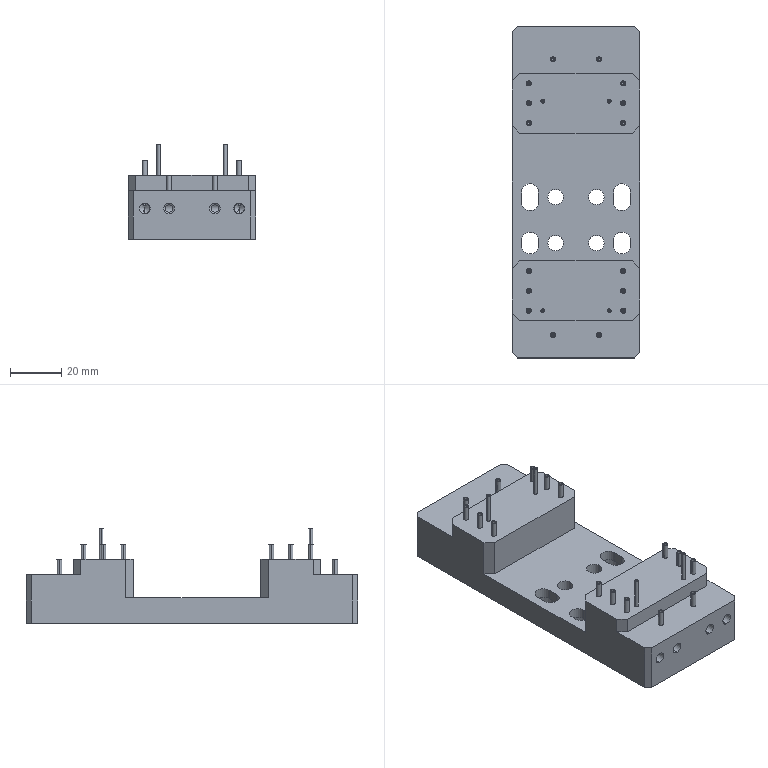Component | SolidWorks | 6.11-1937032103-0-1 | 21 solids | 451 faces | volume 97355 mm3 | cylinder 266 | cone 93 | plane 92 | commonest cylinder face diameters 2 x64 1 x40 1.4 x32 3 x22 4.2 x20 4 x20 1.5 x16 3.3 x12 | material 45#